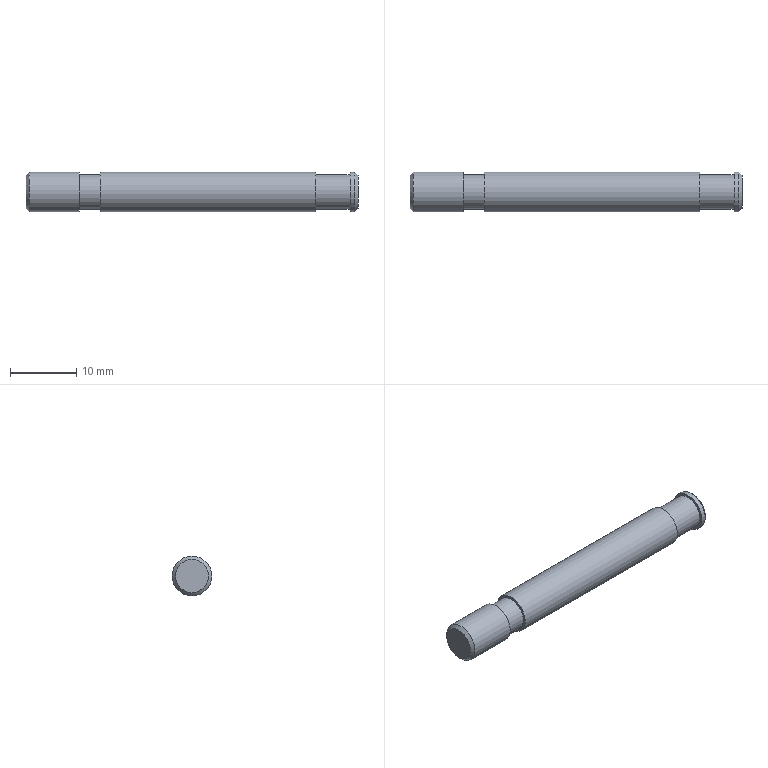Component | NX | FIX_STUD | 1 solid | 13 faces | box 50 x 6 x 6 mm | volume 1349 mm3 | plane 6 | cylinder 5 | cone 2 | commonest cylinder face diameters 6 x3 5.188 x2
STEP:
#1=CARTESIAN_POINT('',(0.,0.,0.));
#2=DIRECTION('',(0.,0.,1.));
#3=DIRECTION('',(1.,0.,0.));
#4=AXIS2_PLACEMENT_3D('',#1,#2,#3);
#5=CARTESIAN_POINT('',(-18.8,-32.,-54.));
#6=VERTEX_POINT('',#5);
#7=CARTESIAN_POINT('',(-18.8,-32.,-57.));
#8=DIRECTION('',(-1.,0.,0.));
#9=DIRECTION('',(0.,0.,1.));
#10=AXIS2_PLACEMENT_3D('',#7,#8,#9);
#11=CIRCLE('',#10,3.);
#12=CARTESIAN_POINT('',(-30.,-32.,-57.));
#13=DIRECTION('',(1.,0.,0.));
#14=DIRECTION('',(0.,0.,1.));
#15=AXIS2_PLACEMENT_3D('',#12,#13,#14);
#16=CYLINDRICAL_SURFACE('',#15,3.);
#17=CARTESIAN_POINT('',(6.283,11.2));
#18=DIRECTION('',(-1.,0.));
#19=VECTOR('',#18,1.);
#20=LINE('',#17,#19);
#21=(GEOMETRIC_REPRESENTATION_CONTEXT(2)PARAMETRIC_REPRESENTATION_CONTEXT()REPRESENTATION_CONTEXT('',''));
#22=DEFINITIONAL_REPRESENTATION('',(#20),#21);
#23=PCURVE('',#16,#22);
#24=CARTESIAN_POINT('',(-18.8,-32.,-57.));
#25=DIRECTION('',(1.,0.,-0.));
#26=DIRECTION('',(0.,-1.,0.));
#27=AXIS2_PLACEMENT_3D('',#24,#25,#26);
#28=PLANE('',#27);
#29=CARTESIAN_POINT('',(0.,-3.));
#30=CARTESIAN_POINT('',(-5.196,-3.));
#31=CARTESIAN_POINT('',(-2.598,1.5));
#32=CARTESIAN_POINT('',(-0.,6.));
#33=CARTESIAN_POINT('',(2.598,1.5));
#34=CARTESIAN_POINT('',(5.196,-3.));
#35=CARTESIAN_POINT('',(0.,-3.));
#36=(BOUNDED_CURVE()B_SPLINE_CURVE(2,(#29,#30,#31,#32,#33,#34,#35),.UNSPECIFIED.,.T.,.F.)B_SPLINE_CURVE_WITH_KNOTS((1,2,2,2,2,1),(-2.094,0.,2.094,4.189,6.283,8.378),.UNSPECIFIED.)CURVE()GEOMETRIC_REPRESENTATION_ITEM()RATIONAL_B_SPLINE_CURVE((1.,0.5,1.,0.5,1.,0.5,1.))REPRESENTATION_ITEM(''));
#37=(GEOMETRIC_REPRESENTATION_CONTEXT(2)PARAMETRIC_REPRESENTATION_CONTEXT()REPRESENTATION_CONTEXT('',''));
#38=DEFINITIONAL_REPRESENTATION('',(#36),#37);
#39=PCURVE('',#28,#38);
#40=SURFACE_CURVE('',#11,(#23,#39),.PCURVE_S1.);
#41=EDGE_CURVE('',#6,#6,#40,.T.);
#42=ORIENTED_EDGE('',*,*,#41,.F.);
#43=CARTESIAN_POINT('',(13.6,-32.,-54.));
#44=VERTEX_POINT('',#43);
#45=CARTESIAN_POINT('',(-18.8,-32.,-54.));
#46=CARTESIAN_POINT('',(13.6,-32.,-54.));
#47=B_SPLINE_CURVE_WITH_KNOTS('',1,(#45,#46),.UNSPECIFIED.,.F.,.F.,(2,2),(11.2,43.6),.PIECEWISE_BEZIER_KNOTS.);
#48=CARTESIAN_POINT('',(6.283,0.));
#49=DIRECTION('',(0.,1.));
#50=VECTOR('',#49,1.);
#51=LINE('',#48,#50);
#52=(GEOMETRIC_REPRESENTATION_CONTEXT(2)PARAMETRIC_REPRESENTATION_CONTEXT()REPRESENTATION_CONTEXT('',''));
#53=DEFINITIONAL_REPRESENTATION('',(#51),#52);
#54=PCURVE('',#16,#53);
#55=CARTESIAN_POINT('',(0.,0.));
#56=DIRECTION('',(0.,1.));
#57=VECTOR('',#56,1.);
#58=LINE('',#55,#57);
#59=(GEOMETRIC_REPRESENTATION_CONTEXT(2)PARAMETRIC_REPRESENTATION_CONTEXT()REPRESENTATION_CONTEXT('',''));
#60=DEFINITIONAL_REPRESENTATION('',(#58),#59);
#61=PCURVE('',#16,#60);
#62=SEAM_CURVE('',#47,(#54,#61),.PCURVE_S1.);
#63=EDGE_CURVE('',#6,#44,#62,.T.);
#64=ORIENTED_EDGE('',*,*,#63,.T.);
#65=CARTESIAN_POINT('',(13.6,-32.,-57.));
#66=DIRECTION('',(-1.,0.,0.));
#67=DIRECTION('',(0.,0.,1.));
#68=AXIS2_PLACEMENT_3D('',#65,#66,#67);
#69=CIRCLE('',#68,3.);
#70=CARTESIAN_POINT('',(6.283,43.6));
#71=DIRECTION('',(-1.,0.));
#72=VECTOR('',#71,1.);
#73=LINE('',#70,#72);
#74=(GEOMETRIC_REPRESENTATION_CONTEXT(2)PARAMETRIC_REPRESENTATION_CONTEXT()REPRESENTATION_CONTEXT('',''));
#75=DEFINITIONAL_REPRESENTATION('',(#73),#74);
#76=PCURVE('',#16,#75);
#77=CARTESIAN_POINT('',(13.6,-32.,-57.));
#78=DIRECTION('',(1.,0.,-0.));
#79=DIRECTION('',(0.,-1.,0.));
#80=AXIS2_PLACEMENT_3D('',#77,#78,#79);
#81=PLANE('',#80);
#82=CARTESIAN_POINT('',(0.,-3.));
#83=CARTESIAN_POINT('',(-5.196,-3.));
#84=CARTESIAN_POINT('',(-2.598,1.5));
#85=CARTESIAN_POINT('',(-0.,6.));
#86=CARTESIAN_POINT('',(2.598,1.5));
#87=CARTESIAN_POINT('',(5.196,-3.));
#88=CARTESIAN_POINT('',(0.,-3.));
#89=(BOUNDED_CURVE()B_SPLINE_CURVE(2,(#82,#83,#84,#85,#86,#87,#88),.UNSPECIFIED.,.T.,.F.)B_SPLINE_CURVE_WITH_KNOTS((1,2,2,2,2,1),(-2.094,0.,2.094,4.189,6.283,8.378),.UNSPECIFIED.)CURVE()GEOMETRIC_REPRESENTATION_ITEM()RATIONAL_B_SPLINE_CURVE((1.,0.5,1.,0.5,1.,0.5,1.))REPRESENTATION_ITEM(''));
#90=(GEOMETRIC_REPRESENTATION_CONTEXT(2)PARAMETRIC_REPRESENTATION_CONTEXT()REPRESENTATION_CONTEXT('',''));
#91=DEFINITIONAL_REPRESENTATION('',(#89),#90);
#92=PCURVE('',#81,#91);
#93=SURFACE_CURVE('',#69,(#76,#92),.PCURVE_S1.);
#94=EDGE_CURVE('',#44,#44,#93,.T.);
#95=ORIENTED_EDGE('',*,*,#94,.T.);
#96=ORIENTED_EDGE('',*,*,#63,.F.);
#97=EDGE_LOOP('',(#42,#64,#95,#96));
#98=FACE_BOUND('',#97,.T.);
#99=ADVANCED_FACE('',(#98),#16,.T.);
#100=ORIENTED_EDGE('',*,*,#41,.T.);
#101=EDGE_LOOP('',(#100));
#102=FACE_BOUND('',#101,.T.);
#103=CARTESIAN_POINT('',(-18.8,-32.,-54.406));
#104=VERTEX_POINT('',#103);
#105=CARTESIAN_POINT('',(-18.8,-32.,-57.));
#106=DIRECTION('',(1.,0.,-0.));
#107=DIRECTION('',(0.,0.,1.));
#108=AXIS2_PLACEMENT_3D('',#105,#106,#107);
#109=CIRCLE('',#108,2.594);
#110=CARTESIAN_POINT('',(0.,0.));
#111=DIRECTION('',(0.,-1.));
#112=AXIS2_PLACEMENT_2D('',#110,#111);
#113=CIRCLE('',#112,2.594);
#114=(GEOMETRIC_REPRESENTATION_CONTEXT(2)PARAMETRIC_REPRESENTATION_CONTEXT()REPRESENTATION_CONTEXT('',''));
#115=DEFINITIONAL_REPRESENTATION('',(#113),#114);
#116=PCURVE('',#28,#115);
#117=CARTESIAN_POINT('',(-22.,-32.,-57.));
#118=DIRECTION('',(1.,0.,0.));
#119=DIRECTION('',(0.,0.,1.));
#120=AXIS2_PLACEMENT_3D('',#117,#118,#119);
#121=CYLINDRICAL_SURFACE('',#120,2.594);
#122=CARTESIAN_POINT('',(0.,3.2));
#123=DIRECTION('',(1.,0.));
#124=VECTOR('',#123,1.);
#125=LINE('',#122,#124);
#126=(GEOMETRIC_REPRESENTATION_CONTEXT(2)PARAMETRIC_REPRESENTATION_CONTEXT()REPRESENTATION_CONTEXT('',''));
#127=DEFINITIONAL_REPRESENTATION('',(#125),#126);
#128=PCURVE('',#121,#127);
#129=SURFACE_CURVE('',#109,(#116,#128),.PCURVE_S1.);
#130=EDGE_CURVE('',#104,#104,#129,.T.);
#131=ORIENTED_EDGE('',*,*,#130,.T.);
#132=EDGE_LOOP('',(#131));
#133=FACE_BOUND('',#132,.T.);
#134=ADVANCED_FACE('',(#102,#133),#28,.F.);
#135=CARTESIAN_POINT('',(-22.,-32.,-54.));
#136=VERTEX_POINT('',#135);
#137=CARTESIAN_POINT('',(-22.,-32.,-57.));
#138=DIRECTION('',(-1.,0.,0.));
#139=DIRECTION('',(0.,0.,1.));
#140=AXIS2_PLACEMENT_3D('',#137,#138,#139);
#141=CIRCLE('',#140,3.);
#142=CARTESIAN_POINT('',(-22.,-32.,-57.));
#143=DIRECTION('',(1.,0.,0.));
#144=DIRECTION('',(0.,-1.,0.));
#145=AXIS2_PLACEMENT_3D('',#142,#143,#144);
#146=PLANE('',#145);
#147=CARTESIAN_POINT('',(0.,-3.));
#148=CARTESIAN_POINT('',(-5.196,-3.));
#149=CARTESIAN_POINT('',(-2.598,1.5));
#150=CARTESIAN_POINT('',(-0.,6.));
#151=CARTESIAN_POINT('',(2.598,1.5));
#152=CARTESIAN_POINT('',(5.196,-3.));
#153=CARTESIAN_POINT('',(0.,-3.));
#154=(BOUNDED_CURVE()B_SPLINE_CURVE(2,(#147,#148,#149,#150,#151,#152,#153),.UNSPECIFIED.,.T.,.F.)B_SPLINE_CURVE_WITH_KNOTS((1,2,2,2,2,1),(-2.094,0.,2.094,4.189,6.283,8.378),.UNSPECIFIED.)CURVE()GEOMETRIC_REPRESENTATION_ITEM()RATIONAL_B_SPLINE_CURVE((1.,0.5,1.,0.5,1.,0.5,1.))REPRESENTATION_ITEM(''));
#155=(GEOMETRIC_REPRESENTATION_CONTEXT(2)PARAMETRIC_REPRESENTATION_CONTEXT()REPRESENTATION_CONTEXT('',''));
#156=DEFINITIONAL_REPRESENTATION('',(#154),#155);
#157=PCURVE('',#146,#156);
#158=CARTESIAN_POINT('',(-30.,-32.,-57.));
#159=DIRECTION('',(1.,0.,0.));
#160=DIRECTION('',(0.,0.,1.));
#161=AXIS2_PLACEMENT_3D('',#158,#159,#160);
#162=CYLINDRICAL_SURFACE('',#161,3.);
#163=CARTESIAN_POINT('',(6.283,8.));
#164=DIRECTION('',(-1.,0.));
#165=VECTOR('',#164,1.);
#166=LINE('',#163,#165);
#167=(GEOMETRIC_REPRESENTATION_CONTEXT(2)PARAMETRIC_REPRESENTATION_CONTEXT()REPRESENTATION_CONTEXT('',''));
#168=DEFINITIONAL_REPRESENTATION('',(#166),#167);
#169=PCURVE('',#162,#168);
#170=SURFACE_CURVE('',#141,(#157,#169),.PCURVE_S1.);
#171=EDGE_CURVE('',#136,#136,#170,.T.);
#172=ORIENTED_EDGE('',*,*,#171,.F.);
#173=EDGE_LOOP('',(#172));
#174=FACE_BOUND('',#173,.T.);
#175=CARTESIAN_POINT('',(-22.,-32.,-54.406));
#176=VERTEX_POINT('',#175);
#177=CARTESIAN_POINT('',(-22.,-32.,-57.));
#178=DIRECTION('',(1.,0.,0.));
#179=DIRECTION('',(0.,0.,1.));
#180=AXIS2_PLACEMENT_3D('',#177,#178,#179);
#181=CIRCLE('',#180,2.594);
#182=CARTESIAN_POINT('',(0.,0.));
#183=DIRECTION('',(0.,-1.));
#184=AXIS2_PLACEMENT_2D('',#182,#183);
#185=CIRCLE('',#184,2.594);
#186=(GEOMETRIC_REPRESENTATION_CONTEXT(2)PARAMETRIC_REPRESENTATION_CONTEXT()REPRESENTATION_CONTEXT('',''));
#187=DEFINITIONAL_REPRESENTATION('',(#185),#186);
#188=PCURVE('',#146,#187);
#189=CARTESIAN_POINT('',(0.,0.));
#190=DIRECTION('',(1.,0.));
#191=VECTOR('',#190,1.);
#192=LINE('',#189,#191);
#193=(GEOMETRIC_REPRESENTATION_CONTEXT(2)PARAMETRIC_REPRESENTATION_CONTEXT()REPRESENTATION_CONTEXT('',''));
#194=DEFINITIONAL_REPRESENTATION('',(#192),#193);
#195=PCURVE('',#121,#194);
#196=SURFACE_CURVE('',#181,(#188,#195),.PCURVE_S1.);
#197=EDGE_CURVE('',#176,#176,#196,.T.);
#198=ORIENTED_EDGE('',*,*,#197,.F.);
#199=EDGE_LOOP('',(#198));
#200=FACE_BOUND('',#199,.T.);
#201=ADVANCED_FACE('',(#174,#200),#146,.T.);
#202=ORIENTED_EDGE('',*,*,#197,.T.);
#203=CARTESIAN_POINT('',(-22.,-32.,-54.406));
#204=CARTESIAN_POINT('',(-18.8,-32.,-54.406));
#205=B_SPLINE_CURVE_WITH_KNOTS('',1,(#203,#204),.UNSPECIFIED.,.F.,.F.,(2,2),(0.,3.2),.PIECEWISE_BEZIER_KNOTS.);
#206=CARTESIAN_POINT('',(6.283,0.));
#207=DIRECTION('',(0.,1.));
#208=VECTOR('',#207,1.);
#209=LINE('',#206,#208);
#210=(GEOMETRIC_REPRESENTATION_CONTEXT(2)PARAMETRIC_REPRESENTATION_CONTEXT()REPRESENTATION_CONTEXT('',''));
#211=DEFINITIONAL_REPRESENTATION('',(#209),#210);
#212=PCURVE('',#121,#211);
#213=CARTESIAN_POINT('',(0.,0.));
#214=DIRECTION('',(0.,1.));
#215=VECTOR('',#214,1.);
#216=LINE('',#213,#215);
#217=(GEOMETRIC_REPRESENTATION_CONTEXT(2)PARAMETRIC_REPRESENTATION_CONTEXT()REPRESENTATION_CONTEXT('',''));
#218=DEFINITIONAL_REPRESENTATION('',(#216),#217);
#219=PCURVE('',#121,#218);
#220=SEAM_CURVE('',#205,(#212,#219),.PCURVE_S1.);
#221=EDGE_CURVE('',#176,#104,#220,.T.);
#222=ORIENTED_EDGE('',*,*,#221,.T.);
#223=ORIENTED_EDGE('',*,*,#130,.F.);
#224=ORIENTED_EDGE('',*,*,#221,.F.);
#225=EDGE_LOOP('',(#202,#222,#223,#224));
#226=FACE_BOUND('',#225,.T.);
#227=ADVANCED_FACE('',(#226),#121,.T.);
#228=CARTESIAN_POINT('',(-30.,-32.,-59.5));
#229=VERTEX_POINT('',#228);
#230=CARTESIAN_POINT('',(-30.,-32.,-57.));
#231=DIRECTION('',(-1.,0.,0.));
#232=DIRECTION('',(0.,0.,-1.));
#233=AXIS2_PLACEMENT_3D('',#230,#231,#232);
#234=CIRCLE('',#233,2.5);
#235=CARTESIAN_POINT('',(-30.,-32.,-57.));
#236=DIRECTION('',(-1.,0.,0.));
#237=DIRECTION('',(0.,0.,-1.));
#238=AXIS2_PLACEMENT_3D('',#235,#236,#237);
#239=PLANE('',#238);
#240=CARTESIAN_POINT('',(0.,0.));
#241=DIRECTION('',(1.,0.));
#242=AXIS2_PLACEMENT_2D('',#240,#241);
#243=CIRCLE('',#242,2.5);
#244=(GEOMETRIC_REPRESENTATION_CONTEXT(2)PARAMETRIC_REPRESENTATION_CONTEXT()REPRESENTATION_CONTEXT('',''));
#245=DEFINITIONAL_REPRESENTATION('',(#243),#244);
#246=PCURVE('',#239,#245);
#247=CARTESIAN_POINT('',(-29.5,-32.,-57.));
#248=DIRECTION('',(1.,0.,0.));
#249=DIRECTION('',(0.,0.,1.));
#250=AXIS2_PLACEMENT_3D('',#247,#248,#249);
#251=CONICAL_SURFACE('',#250,3.,0.7854);
#252=CARTESIAN_POINT('',(9.425,-0.5));
#253=DIRECTION('',(-1.,0.));
#254=VECTOR('',#253,1.);
#255=LINE('',#252,#254);
#256=(GEOMETRIC_REPRESENTATION_CONTEXT(2)PARAMETRIC_REPRESENTATION_CONTEXT()REPRESENTATION_CONTEXT('',''));
#257=DEFINITIONAL_REPRESENTATION('',(#255),#256);
#258=PCURVE('',#251,#257);
#259=SURFACE_CURVE('',#234,(#246,#258),.PCURVE_S1.);
#260=EDGE_CURVE('',#229,#229,#259,.T.);
#261=ORIENTED_EDGE('',*,*,#260,.T.);
#262=EDGE_LOOP('',(#261));
#263=FACE_BOUND('',#262,.T.);
#264=ADVANCED_FACE('',(#263),#239,.T.);
#265=ORIENTED_EDGE('',*,*,#260,.F.);
#266=CARTESIAN_POINT('',(-29.5,-32.,-60.));
#267=VERTEX_POINT('',#266);
#268=CARTESIAN_POINT('',(-30.,-32.,-59.5));
#269=CARTESIAN_POINT('',(-29.5,-32.,-60.));
#270=B_SPLINE_CURVE_WITH_KNOTS('',1,(#268,#269),.UNSPECIFIED.,.F.,.F.,(2,2),(-0.7071,0.),.PIECEWISE_BEZIER_KNOTS.);
#271=CARTESIAN_POINT('',(9.425,0.));
#272=DIRECTION('',(0.,1.));
#273=VECTOR('',#272,1.);
#274=LINE('',#271,#273);
#275=(GEOMETRIC_REPRESENTATION_CONTEXT(2)PARAMETRIC_REPRESENTATION_CONTEXT()REPRESENTATION_CONTEXT('',''));
#276=DEFINITIONAL_REPRESENTATION('',(#274),#275);
#277=PCURVE('',#251,#276);
#278=CARTESIAN_POINT('',(3.142,0.));
#279=DIRECTION('',(0.,1.));
#280=VECTOR('',#279,1.);
#281=LINE('',#278,#280);
#282=(GEOMETRIC_REPRESENTATION_CONTEXT(2)PARAMETRIC_REPRESENTATION_CONTEXT()REPRESENTATION_CONTEXT('',''));
#283=DEFINITIONAL_REPRESENTATION('',(#281),#282);
#284=PCURVE('',#251,#283);
#285=SEAM_CURVE('',#270,(#277,#284),.PCURVE_S1.);
#286=EDGE_CURVE('',#229,#267,#285,.T.);
#287=ORIENTED_EDGE('',*,*,#286,.T.);
#288=CARTESIAN_POINT('',(-29.5,-32.,-54.));
#289=VERTEX_POINT('',#288);
#290=CARTESIAN_POINT('',(-29.5,-32.,-57.));
#291=DIRECTION('',(1.,0.,0.));
#292=DIRECTION('',(0.,0.,-1.));
#293=AXIS2_PLACEMENT_3D('',#290,#291,#292);
#294=CIRCLE('',#293,3.);
#295=CARTESIAN_POINT('',(3.142,0.));
#296=DIRECTION('',(1.,0.));
#297=VECTOR('',#296,1.);
#298=LINE('',#295,#297);
#299=(GEOMETRIC_REPRESENTATION_CONTEXT(2)PARAMETRIC_REPRESENTATION_CONTEXT()REPRESENTATION_CONTEXT('',''));
#300=DEFINITIONAL_REPRESENTATION('',(#298),#299);
#301=PCURVE('',#251,#300);
#302=CARTESIAN_POINT('',(-3.142,0.5));
#303=DIRECTION('',(1.,0.));
#304=VECTOR('',#303,1.);
#305=LINE('',#302,#304);
#306=(GEOMETRIC_REPRESENTATION_CONTEXT(2)PARAMETRIC_REPRESENTATION_CONTEXT()REPRESENTATION_CONTEXT('',''));
#307=DEFINITIONAL_REPRESENTATION('',(#305),#306);
#308=PCURVE('',#162,#307);
#309=SURFACE_CURVE('',#294,(#301,#308),.PCURVE_S1.);
#310=EDGE_CURVE('',#289,#267,#309,.T.);
#311=ORIENTED_EDGE('',*,*,#310,.F.);
#312=CARTESIAN_POINT('',(-29.5,-32.,-57.));
#313=DIRECTION('',(1.,0.,0.));
#314=DIRECTION('',(0.,0.,-1.));
#315=AXIS2_PLACEMENT_3D('',#312,#313,#314);
#316=CIRCLE('',#315,3.);
#317=CARTESIAN_POINT('',(3.142,0.));
#318=DIRECTION('',(1.,0.));
#319=VECTOR('',#318,1.);
#320=LINE('',#317,#319);
#321=(GEOMETRIC_REPRESENTATION_CONTEXT(2)PARAMETRIC_REPRESENTATION_CONTEXT()REPRESENTATION_CONTEXT('',''));
#322=DEFINITIONAL_REPRESENTATION('',(#320),#321);
#323=PCURVE('',#251,#322);
#324=CARTESIAN_POINT('',(3.142,0.5));
#325=DIRECTION('',(1.,0.));
#326=VECTOR('',#325,1.);
#327=LINE('',#324,#326);
#328=(GEOMETRIC_REPRESENTATION_CONTEXT(2)PARAMETRIC_REPRESENTATION_CONTEXT()REPRESENTATION_CONTEXT('',''));
#329=DEFINITIONAL_REPRESENTATION('',(#327),#328);
#330=PCURVE('',#162,#329);
#331=SURFACE_CURVE('',#316,(#323,#330),.PCURVE_S1.);
#332=EDGE_CURVE('',#267,#289,#331,.T.);
#333=ORIENTED_EDGE('',*,*,#332,.F.);
#334=ORIENTED_EDGE('',*,*,#286,.F.);
#335=EDGE_LOOP('',(#265,#287,#311,#333,#334));
#336=FACE_BOUND('',#335,.T.);
#337=ADVANCED_FACE('',(#336),#251,.T.);
#338=ORIENTED_EDGE('',*,*,#332,.T.);
#339=CARTESIAN_POINT('',(-29.5,-32.,-54.));
#340=CARTESIAN_POINT('',(-22.,-32.,-54.));
#341=B_SPLINE_CURVE_WITH_KNOTS('',1,(#339,#340),.UNSPECIFIED.,.F.,.F.,(2,2),(0.5,8.),.PIECEWISE_BEZIER_KNOTS.);
#342=CARTESIAN_POINT('',(6.283,0.));
#343=DIRECTION('',(0.,1.));
#344=VECTOR('',#343,1.);
#345=LINE('',#342,#344);
#346=(GEOMETRIC_REPRESENTATION_CONTEXT(2)PARAMETRIC_REPRESENTATION_CONTEXT()REPRESENTATION_CONTEXT('',''));
#347=DEFINITIONAL_REPRESENTATION('',(#345),#346);
#348=PCURVE('',#162,#347);
#349=CARTESIAN_POINT('',(0.,0.));
#350=DIRECTION('',(0.,1.));
#351=VECTOR('',#350,1.);
#352=LINE('',#349,#351);
#353=(GEOMETRIC_REPRESENTATION_CONTEXT(2)PARAMETRIC_REPRESENTATION_CONTEXT()REPRESENTATION_CONTEXT('',''));
#354=DEFINITIONAL_REPRESENTATION('',(#352),#353);
#355=PCURVE('',#162,#354);
#356=SEAM_CURVE('',#341,(#348,#355),.PCURVE_S1.);
#357=EDGE_CURVE('',#289,#136,#356,.T.);
#358=ORIENTED_EDGE('',*,*,#357,.T.);
#359=ORIENTED_EDGE('',*,*,#171,.T.);
#360=ORIENTED_EDGE('',*,*,#357,.F.);
#361=ORIENTED_EDGE('',*,*,#310,.T.);
#362=EDGE_LOOP('',(#338,#358,#359,#360,#361));
#363=FACE_BOUND('',#362,.T.);
#364=ADVANCED_FACE('',(#363),#162,.T.);
#365=CARTESIAN_POINT('',(18.8,-32.,-54.));
#366=VERTEX_POINT('',#365);
#367=CARTESIAN_POINT('',(18.8,-32.,-57.));
#368=DIRECTION('',(-1.,0.,0.));
#369=DIRECTION('',(0.,0.,1.));
#370=AXIS2_PLACEMENT_3D('',#367,#368,#369);
#371=CIRCLE('',#370,3.);
#372=CARTESIAN_POINT('',(18.8,-32.,-57.));
#373=DIRECTION('',(1.,0.,0.));
#374=DIRECTION('',(0.,-1.,0.));
#375=AXIS2_PLACEMENT_3D('',#372,#373,#374);
#376=PLANE('',#375);
#377=CARTESIAN_POINT('',(0.,-3.));
#378=CARTESIAN_POINT('',(-5.196,-3.));
#379=CARTESIAN_POINT('',(-2.598,1.5));
#380=CARTESIAN_POINT('',(-0.,6.));
#381=CARTESIAN_POINT('',(2.598,1.5));
#382=CARTESIAN_POINT('',(5.196,-3.));
#383=CARTESIAN_POINT('',(0.,-3.));
#384=(BOUNDED_CURVE()B_SPLINE_CURVE(2,(#377,#378,#379,#380,#381,#382,#383),.UNSPECIFIED.,.T.,.F.)B_SPLINE_CURVE_WITH_KNOTS((1,2,2,2,2,1),(-2.094,0.,2.094,4.189,6.283,8.378),.UNSPECIFIED.)CURVE()GEOMETRIC_REPRESENTATION_ITEM()RATIONAL_B_SPLINE_CURVE((1.,0.5,1.,0.5,1.,0.5,1.))REPRESENTATION_ITEM(''));
#385=(GEOMETRIC_REPRESENTATION_CONTEXT(2)PARAMETRIC_REPRESENTATION_CONTEXT()REPRESENTATION_CONTEXT('',''));
#386=DEFINITIONAL_REPRESENTATION('',(#384),#385);
#387=PCURVE('',#376,#386);
#388=CARTESIAN_POINT('',(-30.,-32.,-57.));
#389=DIRECTION('',(1.,0.,0.));
#390=DIRECTION('',(0.,0.,1.));
#391=AXIS2_PLACEMENT_3D('',#388,#389,#390);
#392=CYLINDRICAL_SURFACE('',#391,3.);
#393=CARTESIAN_POINT('',(6.283,48.8));
#394=DIRECTION('',(-1.,0.));
#395=VECTOR('',#394,1.);
#396=LINE('',#393,#395);
#397=(GEOMETRIC_REPRESENTATION_CONTEXT(2)PARAMETRIC_REPRESENTATION_CONTEXT()REPRESENTATION_CONTEXT('',''));
#398=DEFINITIONAL_REPRESENTATION('',(#396),#397);
#399=PCURVE('',#392,#398);
#400=SURFACE_CURVE('',#371,(#387,#399),.PCURVE_S1.);
#401=EDGE_CURVE('',#366,#366,#400,.T.);
#402=ORIENTED_EDGE('',*,*,#401,.T.);
#403=EDGE_LOOP('',(#402));
#404=FACE_BOUND('',#403,.T.);
#405=CARTESIAN_POINT('',(18.8,-32.,-54.406));
#406=VERTEX_POINT('',#405);
#407=CARTESIAN_POINT('',(18.8,-32.,-57.));
#408=DIRECTION('',(1.,0.,0.));
#409=DIRECTION('',(0.,0.,1.));
#410=AXIS2_PLACEMENT_3D('',#407,#408,#409);
#411=CIRCLE('',#410,2.594);
#412=CARTESIAN_POINT('',(0.,0.));
#413=DIRECTION('',(0.,-1.));
#414=AXIS2_PLACEMENT_2D('',#412,#413);
#415=CIRCLE('',#414,2.594);
#416=(GEOMETRIC_REPRESENTATION_CONTEXT(2)PARAMETRIC_REPRESENTATION_CONTEXT()REPRESENTATION_CONTEXT('',''));
#417=DEFINITIONAL_REPRESENTATION('',(#415),#416);
#418=PCURVE('',#376,#417);
#419=CARTESIAN_POINT('',(13.6,-32.,-57.));
#420=DIRECTION('',(1.,0.,0.));
#421=DIRECTION('',(0.,0.,1.));
#422=AXIS2_PLACEMENT_3D('',#419,#420,#421);
#423=CYLINDRICAL_SURFACE('',#422,2.594);
#424=CARTESIAN_POINT('',(0.,5.2));
#425=DIRECTION('',(1.,0.));
#426=VECTOR('',#425,1.);
#427=LINE('',#424,#426);
#428=(GEOMETRIC_REPRESENTATION_CONTEXT(2)PARAMETRIC_REPRESENTATION_CONTEXT()REPRESENTATION_CONTEXT('',''));
#429=DEFINITIONAL_REPRESENTATION('',(#427),#428);
#430=PCURVE('',#423,#429);
#431=SURFACE_CURVE('',#411,(#418,#430),.PCURVE_S1.);
#432=EDGE_CURVE('',#406,#406,#431,.T.);
#433=ORIENTED_EDGE('',*,*,#432,.T.);
#434=EDGE_LOOP('',(#433));
#435=FACE_BOUND('',#434,.T.);
#436=ADVANCED_FACE('',(#404,#435),#376,.F.);
#437=ORIENTED_EDGE('',*,*,#94,.F.);
#438=EDGE_LOOP('',(#437));
#439=FACE_BOUND('',#438,.T.);
#440=CARTESIAN_POINT('',(13.6,-32.,-54.406));
#441=VERTEX_POINT('',#440);
#442=CARTESIAN_POINT('',(13.6,-32.,-57.));
#443=DIRECTION('',(1.,0.,-0.));
#444=DIRECTION('',(0.,0.,1.));
#445=AXIS2_PLACEMENT_3D('',#442,#443,#444);
#446=CIRCLE('',#445,2.594);
#447=CARTESIAN_POINT('',(0.,0.));
#448=DIRECTION('',(0.,-1.));
#449=AXIS2_PLACEMENT_2D('',#447,#448);
#450=CIRCLE('',#449,2.594);
#451=(GEOMETRIC_REPRESENTATION_CONTEXT(2)PARAMETRIC_REPRESENTATION_CONTEXT()REPRESENTATION_CONTEXT('',''));
#452=DEFINITIONAL_REPRESENTATION('',(#450),#451);
#453=PCURVE('',#81,#452);
#454=CARTESIAN_POINT('',(0.,0.));
#455=DIRECTION('',(1.,0.));
#456=VECTOR('',#455,1.);
#457=LINE('',#454,#456);
#458=(GEOMETRIC_REPRESENTATION_CONTEXT(2)PARAMETRIC_REPRESENTATION_CONTEXT()REPRESENTATION_CONTEXT('',''));
#459=DEFINITIONAL_REPRESENTATION('',(#457),#458);
#460=PCURVE('',#423,#459);
#461=SURFACE_CURVE('',#446,(#453,#460),.PCURVE_S1.);
#462=EDGE_CURVE('',#441,#441,#461,.T.);
#463=ORIENTED_EDGE('',*,*,#462,.F.);
#464=EDGE_LOOP('',(#463));
#465=FACE_BOUND('',#464,.T.);
#466=ADVANCED_FACE('',(#439,#465),#81,.T.);
#467=ORIENTED_EDGE('',*,*,#462,.T.);
#468=CARTESIAN_POINT('',(13.6,-32.,-54.406));
#469=CARTESIAN_POINT('',(18.8,-32.,-54.406));
#470=B_SPLINE_CURVE_WITH_KNOTS('',1,(#468,#469),.UNSPECIFIED.,.F.,.F.,(2,2),(0.,5.2),.PIECEWISE_BEZIER_KNOTS.);
#471=CARTESIAN_POINT('',(6.283,0.));
#472=DIRECTION('',(0.,1.));
#473=VECTOR('',#472,1.);
#474=LINE('',#471,#473);
#475=(GEOMETRIC_REPRESENTATION_CONTEXT(2)PARAMETRIC_REPRESENTATION_CONTEXT()REPRESENTATION_CONTEXT('',''));
#476=DEFINITIONAL_REPRESENTATION('',(#474),#475);
#477=PCURVE('',#423,#476);
#478=CARTESIAN_POINT('',(0.,0.));
#479=DIRECTION('',(0.,1.));
#480=VECTOR('',#479,1.);
#481=LINE('',#478,#480);
#482=(GEOMETRIC_REPRESENTATION_CONTEXT(2)PARAMETRIC_REPRESENTATION_CONTEXT()REPRESENTATION_CONTEXT('',''));
#483=DEFINITIONAL_REPRESENTATION('',(#481),#482);
#484=PCURVE('',#423,#483);
#485=SEAM_CURVE('',#470,(#477,#484),.PCURVE_S1.);
#486=EDGE_CURVE('',#441,#406,#485,.T.);
#487=ORIENTED_EDGE('',*,*,#486,.T.);
#488=ORIENTED_EDGE('',*,*,#432,.F.);
#489=ORIENTED_EDGE('',*,*,#486,.F.);
#490=EDGE_LOOP('',(#467,#487,#488,#489));
#491=FACE_BOUND('',#490,.T.);
#492=ADVANCED_FACE('',(#491),#423,.T.);
#493=CARTESIAN_POINT('',(20.,-32.,-54.5));
#494=VERTEX_POINT('',#493);
#495=CARTESIAN_POINT('',(20.,-32.,-57.));
#496=DIRECTION('',(1.,0.,0.));
#497=DIRECTION('',(0.,0.,1.));
#498=AXIS2_PLACEMENT_3D('',#495,#496,#497);
#499=CIRCLE('',#498,2.5);
#500=CARTESIAN_POINT('',(20.,-32.,-57.));
#501=DIRECTION('',(1.,0.,0.));
#502=DIRECTION('',(0.,0.,1.));
#503=AXIS2_PLACEMENT_3D('',#500,#501,#502);
#504=PLANE('',#503);
#505=CARTESIAN_POINT('',(0.,0.));
#506=DIRECTION('',(1.,0.));
#507=AXIS2_PLACEMENT_2D('',#505,#506);
#508=CIRCLE('',#507,2.5);
#509=(GEOMETRIC_REPRESENTATION_CONTEXT(2)PARAMETRIC_REPRESENTATION_CONTEXT()REPRESENTATION_CONTEXT('',''));
#510=DEFINITIONAL_REPRESENTATION('',(#508),#509);
#511=PCURVE('',#504,#510);
#512=CARTESIAN_POINT('',(19.5,-32.,-57.));
#513=DIRECTION('',(-1.,0.,0.));
#514=DIRECTION('',(0.,0.,-1.));
#515=AXIS2_PLACEMENT_3D('',#512,#513,#514);
#516=CONICAL_SURFACE('',#515,3.,0.7854);
#517=CARTESIAN_POINT('',(9.425,-0.5));
#518=DIRECTION('',(-1.,0.));
#519=VECTOR('',#518,1.);
#520=LINE('',#517,#519);
#521=(GEOMETRIC_REPRESENTATION_CONTEXT(2)PARAMETRIC_REPRESENTATION_CONTEXT()REPRESENTATION_CONTEXT('',''));
#522=DEFINITIONAL_REPRESENTATION('',(#520),#521);
#523=PCURVE('',#516,#522);
#524=SURFACE_CURVE('',#499,(#511,#523),.PCURVE_S1.);
#525=EDGE_CURVE('',#494,#494,#524,.T.);
#526=ORIENTED_EDGE('',*,*,#525,.T.);
#527=EDGE_LOOP('',(#526));
#528=FACE_BOUND('',#527,.T.);
#529=ADVANCED_FACE('',(#528),#504,.T.);
#530=ORIENTED_EDGE('',*,*,#525,.F.);
#531=CARTESIAN_POINT('',(19.5,-32.,-54.));
#532=VERTEX_POINT('',#531);
#533=CARTESIAN_POINT('',(20.,-32.,-54.5));
#534=CARTESIAN_POINT('',(19.5,-32.,-54.));
#535=B_SPLINE_CURVE_WITH_KNOTS('',1,(#533,#534),.UNSPECIFIED.,.F.,.F.,(2,2),(-0.7071,0.),.PIECEWISE_BEZIER_KNOTS.);
#536=CARTESIAN_POINT('',(9.425,0.));
#537=DIRECTION('',(0.,1.));
#538=VECTOR('',#537,1.);
#539=LINE('',#536,#538);
#540=(GEOMETRIC_REPRESENTATION_CONTEXT(2)PARAMETRIC_REPRESENTATION_CONTEXT()REPRESENTATION_CONTEXT('',''));
#541=DEFINITIONAL_REPRESENTATION('',(#539),#540);
#542=PCURVE('',#516,#541);
#543=CARTESIAN_POINT('',(3.142,0.));
#544=DIRECTION('',(0.,1.));
#545=VECTOR('',#544,1.);
#546=LINE('',#543,#545);
#547=(GEOMETRIC_REPRESENTATION_CONTEXT(2)PARAMETRIC_REPRESENTATION_CONTEXT()REPRESENTATION_CONTEXT('',''));
#548=DEFINITIONAL_REPRESENTATION('',(#546),#547);
#549=PCURVE('',#516,#548);
#550=SEAM_CURVE('',#535,(#542,#549),.PCURVE_S1.);
#551=EDGE_CURVE('',#494,#532,#550,.T.);
#552=ORIENTED_EDGE('',*,*,#551,.T.);
#553=CARTESIAN_POINT('',(19.5,-32.,-57.));
#554=DIRECTION('',(-1.,0.,0.));
#555=DIRECTION('',(0.,0.,1.));
#556=AXIS2_PLACEMENT_3D('',#553,#554,#555);
#557=CIRCLE('',#556,3.);
#558=CARTESIAN_POINT('',(3.142,0.));
#559=DIRECTION('',(1.,0.));
#560=VECTOR('',#559,1.);
#561=LINE('',#558,#560);
#562=(GEOMETRIC_REPRESENTATION_CONTEXT(2)PARAMETRIC_REPRESENTATION_CONTEXT()REPRESENTATION_CONTEXT('',''));
#563=DEFINITIONAL_REPRESENTATION('',(#561),#562);
#564=PCURVE('',#516,#563);
#565=CARTESIAN_POINT('',(6.283,49.5));
#566=DIRECTION('',(-1.,0.));
#567=VECTOR('',#566,1.);
#568=LINE('',#565,#567);
#569=(GEOMETRIC_REPRESENTATION_CONTEXT(2)PARAMETRIC_REPRESENTATION_CONTEXT()REPRESENTATION_CONTEXT('',''));
#570=DEFINITIONAL_REPRESENTATION('',(#568),#569);
#571=PCURVE('',#392,#570);
#572=SURFACE_CURVE('',#557,(#564,#571),.PCURVE_S1.);
#573=EDGE_CURVE('',#532,#532,#572,.T.);
#574=ORIENTED_EDGE('',*,*,#573,.F.);
#575=ORIENTED_EDGE('',*,*,#551,.F.);
#576=EDGE_LOOP('',(#530,#552,#574,#575));
#577=FACE_BOUND('',#576,.T.);
#578=ADVANCED_FACE('',(#577),#516,.T.);
#579=ORIENTED_EDGE('',*,*,#401,.F.);
#580=CARTESIAN_POINT('',(18.8,-32.,-54.));
#581=CARTESIAN_POINT('',(19.5,-32.,-54.));
#582=B_SPLINE_CURVE_WITH_KNOTS('',1,(#580,#581),.UNSPECIFIED.,.F.,.F.,(2,2),(48.8,49.5),.PIECEWISE_BEZIER_KNOTS.);
#583=CARTESIAN_POINT('',(6.283,0.));
#584=DIRECTION('',(0.,1.));
#585=VECTOR('',#584,1.);
#586=LINE('',#583,#585);
#587=(GEOMETRIC_REPRESENTATION_CONTEXT(2)PARAMETRIC_REPRESENTATION_CONTEXT()REPRESENTATION_CONTEXT('',''));
#588=DEFINITIONAL_REPRESENTATION('',(#586),#587);
#589=PCURVE('',#392,#588);
#590=CARTESIAN_POINT('',(0.,0.));
#591=DIRECTION('',(0.,1.));
#592=VECTOR('',#591,1.);
#593=LINE('',#590,#592);
#594=(GEOMETRIC_REPRESENTATION_CONTEXT(2)PARAMETRIC_REPRESENTATION_CONTEXT()REPRESENTATION_CONTEXT('',''));
#595=DEFINITIONAL_REPRESENTATION('',(#593),#594);
#596=PCURVE('',#392,#595);
#597=SEAM_CURVE('',#582,(#589,#596),.PCURVE_S1.);
#598=EDGE_CURVE('',#366,#532,#597,.T.);
#599=ORIENTED_EDGE('',*,*,#598,.T.);
#600=ORIENTED_EDGE('',*,*,#573,.T.);
#601=ORIENTED_EDGE('',*,*,#598,.F.);
#602=EDGE_LOOP('',(#579,#599,#600,#601));
#603=FACE_BOUND('',#602,.T.);
#604=ADVANCED_FACE('',(#603),#392,.T.);
#605=CLOSED_SHELL('',(#99,#134,#201,#227,#264,#337,#364,#436,#466,#492,#529,#578,#604));
#606=MANIFOLD_SOLID_BREP('',#605);
#607=(LENGTH_UNIT()NAMED_UNIT(*)SI_UNIT(.MILLI.,.METRE.));
#608=UNCERTAINTY_MEASURE_WITH_UNIT(LENGTH_MEASURE(0.00001),#607,'','');
#609=(NAMED_UNIT(*)PLANE_ANGLE_UNIT()SI_UNIT($,.RADIAN.));
#610=(NAMED_UNIT(*)SI_UNIT($,.STERADIAN.)SOLID_ANGLE_UNIT());
#611=(GEOMETRIC_REPRESENTATION_CONTEXT(3)GLOBAL_UNCERTAINTY_ASSIGNED_CONTEXT((#608))GLOBAL_UNIT_ASSIGNED_CONTEXT((#607,#609,#610))REPRESENTATION_CONTEXT('',''));
#612=ADVANCED_BREP_SHAPE_REPRESENTATION('',(#4,#606),#611);